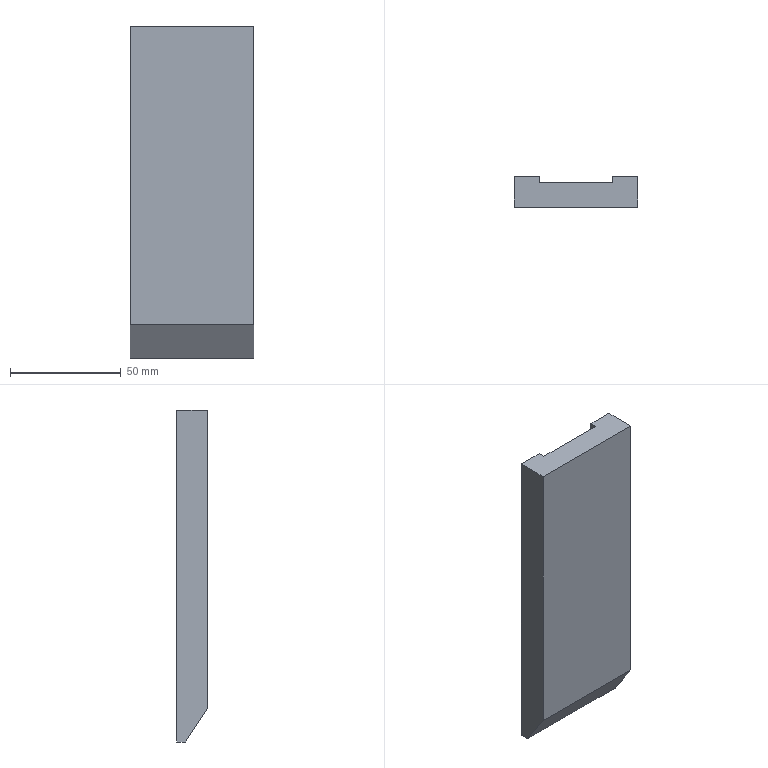Component | SolidWorks | CHEN123-AA-16-1 | 1 solid | 11 faces | box 56 x 14 x 150 mm | volume 98550 mm3 | plane 11
build123d program:
from build123d import *

# Parameters (mm, degrees)
SKETCH1_W           = 150
SKETCH1_H           = 56
BOSS_EXTRUDE1_DEPTH = 14
CUT_EXTRUDE1_DEPTH  = 95.641
SKETCH3_W           = 197.23
SKETCH3_H           = 33
CUT_EXTRUDE2_DEPTH  = 3


with BuildPart() as part:
    # Sketch1 → Boss-Extrude1 (new body)
    with BuildSketch(Plane.XY):
        Rectangle(SKETCH1_W, SKETCH1_H)
    extrude(amount=BOSS_EXTRUDE1_DEPTH)

    # Sketch2 → Cut-Extrude1 (cut, through all)
    with BuildSketch(Plane(origin=(0, 28, 0), x_dir=(1, 0, 0), z_dir=(0, 1, 0))):
        Polygon((-75, -14), (-75, -4), (-60, -14), align=None)
    extrude(amount=-CUT_EXTRUDE1_DEPTH, mode=Mode.SUBTRACT)

    # Sketch3 → Cut-Extrude2 (cut)
    with BuildSketch(Plane(origin=(0, 0, 0), x_dir=(-1, 0, 0), z_dir=(0, 0, -1))):
        Rectangle(SKETCH3_W, SKETCH3_H)
    extrude(amount=-CUT_EXTRUDE2_DEPTH, mode=Mode.SUBTRACT)


solid = part.part

# Placed as in the assembly
solid = solid.moved(Location((-0.0005, 34.001, -345), (90, 0, 90)))
STEP:
#1=CARTESIAN_POINT('',(-0.6496,1.339,-16.535));
#2=VERTEX_POINT('',#1);
#3=CARTESIAN_POINT('',(-0.6496,1.339,-10.63));
#4=VERTEX_POINT('',#3);
#5=CARTESIAN_POINT('',(-0.6496,1.339,-13.583));
#6=DIRECTION('',(0.,0.,1.));
#7=VECTOR('',#6,39.37);
#8=LINE('',#5,#7);
#9=EDGE_CURVE('',#2,#4,#8,.T.);
#10=ORIENTED_EDGE('',*,*,#9,.F.);
#11=CARTESIAN_POINT('',(-1.102,1.339,-16.535));
#12=VERTEX_POINT('',#11);
#13=CARTESIAN_POINT('',(1.102,1.339,-16.535));
#14=DIRECTION('',(1.,-0.,-0.));
#15=VECTOR('',#14,39.37);
#16=LINE('',#13,#15);
#17=EDGE_CURVE('',#12,#2,#16,.T.);
#18=ORIENTED_EDGE('',*,*,#17,.F.);
#19=CARTESIAN_POINT('',(-1.102,1.339,-10.63));
#20=VERTEX_POINT('',#19);
#21=CARTESIAN_POINT('',(-1.102,1.339,-16.535));
#22=DIRECTION('',(-0.,-0.,-1.));
#23=VECTOR('',#22,39.37);
#24=LINE('',#21,#23);
#25=EDGE_CURVE('',#20,#12,#24,.T.);
#26=ORIENTED_EDGE('',*,*,#25,.F.);
#27=CARTESIAN_POINT('',(1.102,1.339,-10.63));
#28=DIRECTION('',(-1.,0.,0.));
#29=VECTOR('',#28,39.37);
#30=LINE('',#27,#29);
#31=EDGE_CURVE('',#4,#20,#30,.T.);
#32=ORIENTED_EDGE('',*,*,#31,.F.);
#33=EDGE_LOOP('',(#10,#18,#26,#32));
#34=FACE_OUTER_BOUND('',#33,.T.);
#35=CARTESIAN_POINT('',(-0.00001969,1.339,-13.583));
#36=DIRECTION('',(0.,1.,-0.));
#37=DIRECTION('',(-0.,-0.,-1.));
#38=AXIS2_PLACEMENT_3D('',#35,#36,#37);
#39=PLANE('',#38);
#40=ADVANCED_FACE('',(#34),#39,.T.);
#41=CARTESIAN_POINT('',(0.6496,1.221,-10.63));
#42=VERTEX_POINT('',#41);
#43=CARTESIAN_POINT('',(-0.6496,1.221,-10.63));
#44=VERTEX_POINT('',#43);
#45=CARTESIAN_POINT('',(1.102,1.221,-10.63));
#46=DIRECTION('',(-1.,0.,0.));
#47=VECTOR('',#46,39.37);
#48=LINE('',#45,#47);
#49=EDGE_CURVE('',#42,#44,#48,.T.);
#50=ORIENTED_EDGE('',*,*,#49,.T.);
#51=CARTESIAN_POINT('',(-0.6496,0.7874,-10.63));
#52=DIRECTION('',(0.,1.,-0.));
#53=VECTOR('',#52,39.37);
#54=LINE('',#51,#53);
#55=EDGE_CURVE('',#44,#4,#54,.T.);
#56=ORIENTED_EDGE('',*,*,#55,.T.);
#57=ORIENTED_EDGE('',*,*,#31,.T.);
#58=CARTESIAN_POINT('',(-1.102,0.7874,-10.63));
#59=VERTEX_POINT('',#58);
#60=CARTESIAN_POINT('',(-1.102,0.7874,-10.63));
#61=DIRECTION('',(0.,1.,-0.));
#62=VECTOR('',#61,39.37);
#63=LINE('',#60,#62);
#64=EDGE_CURVE('',#59,#20,#63,.T.);
#65=ORIENTED_EDGE('',*,*,#64,.F.);
#66=CARTESIAN_POINT('',(1.102,0.7874,-10.63));
#67=VERTEX_POINT('',#66);
#68=CARTESIAN_POINT('',(1.102,0.7874,-10.63));
#69=DIRECTION('',(-1.,0.,0.));
#70=VECTOR('',#69,39.37);
#71=LINE('',#68,#70);
#72=EDGE_CURVE('',#67,#59,#71,.T.);
#73=ORIENTED_EDGE('',*,*,#72,.F.);
#74=CARTESIAN_POINT('',(1.102,1.339,-10.63));
#75=VERTEX_POINT('',#74);
#76=CARTESIAN_POINT('',(1.102,0.7874,-10.63));
#77=DIRECTION('',(0.,1.,-0.));
#78=VECTOR('',#77,39.37);
#79=LINE('',#76,#78);
#80=EDGE_CURVE('',#67,#75,#79,.T.);
#81=ORIENTED_EDGE('',*,*,#80,.T.);
#82=CARTESIAN_POINT('',(0.6496,1.339,-10.63));
#83=VERTEX_POINT('',#82);
#84=CARTESIAN_POINT('',(1.102,1.339,-10.63));
#85=DIRECTION('',(-1.,0.,0.));
#86=VECTOR('',#85,39.37);
#87=LINE('',#84,#86);
#88=EDGE_CURVE('',#75,#83,#87,.T.);
#89=ORIENTED_EDGE('',*,*,#88,.T.);
#90=CARTESIAN_POINT('',(0.6496,0.7874,-10.63));
#91=DIRECTION('',(-0.,-1.,0.));
#92=VECTOR('',#91,39.37);
#93=LINE('',#90,#92);
#94=EDGE_CURVE('',#83,#42,#93,.T.);
#95=ORIENTED_EDGE('',*,*,#94,.T.);
#96=EDGE_LOOP('',(#50,#56,#57,#65,#73,#81,#89,#95));
#97=FACE_OUTER_BOUND('',#96,.T.);
#98=CARTESIAN_POINT('',(1.102,0.7874,-10.63));
#99=DIRECTION('',(-0.,-0.,-1.));
#100=DIRECTION('',(-0.,-1.,0.));
#101=AXIS2_PLACEMENT_3D('',#98,#99,#100);
#102=PLANE('',#101);
#103=ADVANCED_FACE('',(#97),#102,.F.);
#104=CARTESIAN_POINT('',(-1.102,1.181,-16.535));
#105=VERTEX_POINT('',#104);
#106=CARTESIAN_POINT('',(-1.102,0.7874,-16.535));
#107=DIRECTION('',(0.,1.,-0.));
#108=VECTOR('',#107,39.37);
#109=LINE('',#106,#108);
#110=EDGE_CURVE('',#105,#12,#109,.T.);
#111=ORIENTED_EDGE('',*,*,#110,.F.);
#112=CARTESIAN_POINT('',(-1.102,0.7874,-15.945));
#113=VERTEX_POINT('',#112);
#114=CARTESIAN_POINT('',(-1.102,1.181,-16.535));
#115=DIRECTION('',(-0.,0.5547,-0.8321));
#116=VECTOR('',#115,39.37);
#117=LINE('',#114,#116);
#118=EDGE_CURVE('',#113,#105,#117,.T.);
#119=ORIENTED_EDGE('',*,*,#118,.F.);
#120=CARTESIAN_POINT('',(-1.102,0.7874,-16.535));
#121=DIRECTION('',(-0.,-0.,-1.));
#122=VECTOR('',#121,39.37);
#123=LINE('',#120,#122);
#124=EDGE_CURVE('',#59,#113,#123,.T.);
#125=ORIENTED_EDGE('',*,*,#124,.F.);
#126=ORIENTED_EDGE('',*,*,#64,.T.);
#127=ORIENTED_EDGE('',*,*,#25,.T.);
#128=EDGE_LOOP('',(#111,#119,#125,#126,#127));
#129=FACE_OUTER_BOUND('',#128,.T.);
#130=CARTESIAN_POINT('',(-1.102,0.7874,-16.535));
#131=DIRECTION('',(1.,-0.,-0.));
#132=DIRECTION('',(0.,1.,-0.));
#133=AXIS2_PLACEMENT_3D('',#130,#131,#132);
#134=PLANE('',#133);
#135=ADVANCED_FACE('',(#129),#134,.F.);
#136=ORIENTED_EDGE('',*,*,#17,.T.);
#137=CARTESIAN_POINT('',(-0.6496,1.221,-16.535));
#138=VERTEX_POINT('',#137);
#139=CARTESIAN_POINT('',(-0.6496,0.7874,-16.535));
#140=DIRECTION('',(-0.,-1.,0.));
#141=VECTOR('',#140,39.37);
#142=LINE('',#139,#141);
#143=EDGE_CURVE('',#2,#138,#142,.T.);
#144=ORIENTED_EDGE('',*,*,#143,.T.);
#145=CARTESIAN_POINT('',(0.6496,1.221,-16.535));
#146=VERTEX_POINT('',#145);
#147=CARTESIAN_POINT('',(1.102,1.221,-16.535));
#148=DIRECTION('',(1.,-0.,-0.));
#149=VECTOR('',#148,39.37);
#150=LINE('',#147,#149);
#151=EDGE_CURVE('',#138,#146,#150,.T.);
#152=ORIENTED_EDGE('',*,*,#151,.T.);
#153=CARTESIAN_POINT('',(0.6496,1.339,-16.535));
#154=VERTEX_POINT('',#153);
#155=CARTESIAN_POINT('',(0.6496,0.7874,-16.535));
#156=DIRECTION('',(0.,1.,-0.));
#157=VECTOR('',#156,39.37);
#158=LINE('',#155,#157);
#159=EDGE_CURVE('',#146,#154,#158,.T.);
#160=ORIENTED_EDGE('',*,*,#159,.T.);
#161=CARTESIAN_POINT('',(1.102,1.339,-16.535));
#162=VERTEX_POINT('',#161);
#163=CARTESIAN_POINT('',(1.102,1.339,-16.535));
#164=DIRECTION('',(1.,-0.,-0.));
#165=VECTOR('',#164,39.37);
#166=LINE('',#163,#165);
#167=EDGE_CURVE('',#154,#162,#166,.T.);
#168=ORIENTED_EDGE('',*,*,#167,.T.);
#169=CARTESIAN_POINT('',(1.102,1.181,-16.535));
#170=VERTEX_POINT('',#169);
#171=CARTESIAN_POINT('',(1.102,0.7874,-16.535));
#172=DIRECTION('',(0.,1.,-0.));
#173=VECTOR('',#172,39.37);
#174=LINE('',#171,#173);
#175=EDGE_CURVE('',#170,#162,#174,.T.);
#176=ORIENTED_EDGE('',*,*,#175,.F.);
#177=CARTESIAN_POINT('',(1.102,1.181,-16.535));
#178=DIRECTION('',(-1.,0.,0.));
#179=VECTOR('',#178,39.37);
#180=LINE('',#177,#179);
#181=EDGE_CURVE('',#170,#105,#180,.T.);
#182=ORIENTED_EDGE('',*,*,#181,.T.);
#183=ORIENTED_EDGE('',*,*,#110,.T.);
#184=EDGE_LOOP('',(#136,#144,#152,#160,#168,#176,#182,#183));
#185=FACE_OUTER_BOUND('',#184,.T.);
#186=CARTESIAN_POINT('',(1.102,0.7874,-16.535));
#187=DIRECTION('',(0.,0.,1.));
#188=DIRECTION('',(0.,1.,-0.));
#189=AXIS2_PLACEMENT_3D('',#186,#187,#188);
#190=PLANE('',#189);
#191=ADVANCED_FACE('',(#185),#190,.F.);
#192=CARTESIAN_POINT('',(1.102,0.7874,-15.945));
#193=VERTEX_POINT('',#192);
#194=CARTESIAN_POINT('',(1.102,0.7874,-16.535));
#195=DIRECTION('',(0.,0.,1.));
#196=VECTOR('',#195,39.37);
#197=LINE('',#194,#196);
#198=EDGE_CURVE('',#193,#67,#197,.T.);
#199=ORIENTED_EDGE('',*,*,#198,.F.);
#200=CARTESIAN_POINT('',(1.102,1.181,-16.535));
#201=DIRECTION('',(-0.,0.5547,-0.8321));
#202=VECTOR('',#201,39.37);
#203=LINE('',#200,#202);
#204=EDGE_CURVE('',#193,#170,#203,.T.);
#205=ORIENTED_EDGE('',*,*,#204,.T.);
#206=ORIENTED_EDGE('',*,*,#175,.T.);
#207=CARTESIAN_POINT('',(1.102,1.339,-16.535));
#208=DIRECTION('',(0.,0.,1.));
#209=VECTOR('',#208,39.37);
#210=LINE('',#207,#209);
#211=EDGE_CURVE('',#162,#75,#210,.T.);
#212=ORIENTED_EDGE('',*,*,#211,.T.);
#213=ORIENTED_EDGE('',*,*,#80,.F.);
#214=EDGE_LOOP('',(#199,#205,#206,#212,#213));
#215=FACE_OUTER_BOUND('',#214,.T.);
#216=CARTESIAN_POINT('',(1.102,0.7874,-16.535));
#217=DIRECTION('',(-1.,0.,0.));
#218=DIRECTION('',(-0.,-1.,0.));
#219=AXIS2_PLACEMENT_3D('',#216,#217,#218);
#220=PLANE('',#219);
#221=ADVANCED_FACE('',(#215),#220,.F.);
#222=ORIENTED_EDGE('',*,*,#124,.T.);
#223=CARTESIAN_POINT('',(1.102,0.7874,-15.945));
#224=DIRECTION('',(-1.,0.,0.));
#225=VECTOR('',#224,39.37);
#226=LINE('',#223,#225);
#227=EDGE_CURVE('',#193,#113,#226,.T.);
#228=ORIENTED_EDGE('',*,*,#227,.F.);
#229=ORIENTED_EDGE('',*,*,#198,.T.);
#230=ORIENTED_EDGE('',*,*,#72,.T.);
#231=EDGE_LOOP('',(#222,#228,#229,#230));
#232=FACE_OUTER_BOUND('',#231,.T.);
#233=CARTESIAN_POINT('',(-0.00001969,0.7874,-13.583));
#234=DIRECTION('',(0.,1.,-0.));
#235=DIRECTION('',(-0.,-0.,-1.));
#236=AXIS2_PLACEMENT_3D('',#233,#234,#235);
#237=PLANE('',#236);
#238=ADVANCED_FACE('',(#232),#237,.F.);
#239=CARTESIAN_POINT('',(0.6496,1.339,-13.583));
#240=DIRECTION('',(-0.,-0.,-1.));
#241=VECTOR('',#240,39.37);
#242=LINE('',#239,#241);
#243=EDGE_CURVE('',#83,#154,#242,.T.);
#244=ORIENTED_EDGE('',*,*,#243,.F.);
#245=ORIENTED_EDGE('',*,*,#88,.F.);
#246=ORIENTED_EDGE('',*,*,#211,.F.);
#247=ORIENTED_EDGE('',*,*,#167,.F.);
#248=EDGE_LOOP('',(#244,#245,#246,#247));
#249=FACE_OUTER_BOUND('',#248,.T.);
#250=CARTESIAN_POINT('',(-0.00001969,1.339,-13.583));
#251=DIRECTION('',(0.,1.,-0.));
#252=DIRECTION('',(-0.,-0.,-1.));
#253=AXIS2_PLACEMENT_3D('',#250,#251,#252);
#254=PLANE('',#253);
#255=ADVANCED_FACE('',(#249),#254,.T.);
#256=ORIENTED_EDGE('',*,*,#118,.T.);
#257=ORIENTED_EDGE('',*,*,#181,.F.);
#258=ORIENTED_EDGE('',*,*,#204,.F.);
#259=ORIENTED_EDGE('',*,*,#227,.T.);
#260=EDGE_LOOP('',(#256,#257,#258,#259));
#261=FACE_OUTER_BOUND('',#260,.T.);
#262=CARTESIAN_POINT('',(1.102,1.181,-16.535));
#263=DIRECTION('',(0.,0.8321,0.5547));
#264=DIRECTION('',(-0.,0.5547,-0.8321));
#265=AXIS2_PLACEMENT_3D('',#262,#263,#264);
#266=PLANE('',#265);
#267=ADVANCED_FACE('',(#261),#266,.F.);
#268=CARTESIAN_POINT('',(0.6496,1.221,-17.465));
#269=DIRECTION('',(-0.,-0.,-1.));
#270=VECTOR('',#269,39.37);
#271=LINE('',#268,#270);
#272=EDGE_CURVE('',#42,#146,#271,.T.);
#273=ORIENTED_EDGE('',*,*,#272,.T.);
#274=ORIENTED_EDGE('',*,*,#151,.F.);
#275=CARTESIAN_POINT('',(-0.6496,1.221,-17.465));
#276=DIRECTION('',(0.,0.,1.));
#277=VECTOR('',#276,39.37);
#278=LINE('',#275,#277);
#279=EDGE_CURVE('',#138,#44,#278,.T.);
#280=ORIENTED_EDGE('',*,*,#279,.T.);
#281=ORIENTED_EDGE('',*,*,#49,.F.);
#282=EDGE_LOOP('',(#273,#274,#280,#281));
#283=FACE_OUTER_BOUND('',#282,.T.);
#284=CARTESIAN_POINT('',(-0.00001969,1.221,-13.583));
#285=DIRECTION('',(-0.,-1.,0.));
#286=DIRECTION('',(0.,0.,1.));
#287=AXIS2_PLACEMENT_3D('',#284,#285,#286);
#288=PLANE('',#287);
#289=ADVANCED_FACE('',(#283),#288,.F.);
#290=ORIENTED_EDGE('',*,*,#279,.F.);
#291=ORIENTED_EDGE('',*,*,#143,.F.);
#292=ORIENTED_EDGE('',*,*,#9,.T.);
#293=ORIENTED_EDGE('',*,*,#55,.F.);
#294=EDGE_LOOP('',(#290,#291,#292,#293));
#295=FACE_OUTER_BOUND('',#294,.T.);
#296=CARTESIAN_POINT('',(-0.6496,1.221,-17.465));
#297=DIRECTION('',(-1.,0.,0.));
#298=DIRECTION('',(-0.,-0.,-1.));
#299=AXIS2_PLACEMENT_3D('',#296,#297,#298);
#300=PLANE('',#299);
#301=ADVANCED_FACE('',(#295),#300,.F.);
#302=ORIENTED_EDGE('',*,*,#243,.T.);
#303=ORIENTED_EDGE('',*,*,#159,.F.);
#304=ORIENTED_EDGE('',*,*,#272,.F.);
#305=ORIENTED_EDGE('',*,*,#94,.F.);
#306=EDGE_LOOP('',(#302,#303,#304,#305));
#307=FACE_OUTER_BOUND('',#306,.T.);
#308=CARTESIAN_POINT('',(0.6496,1.221,-17.465));
#309=DIRECTION('',(1.,-0.,-0.));
#310=DIRECTION('',(0.,0.,1.));
#311=AXIS2_PLACEMENT_3D('',#308,#309,#310);
#312=PLANE('',#311);
#313=ADVANCED_FACE('',(#307),#312,.F.);
#314=CLOSED_SHELL('',(#40,#103,#135,#191,#221,#238,#255,#267,#289,#301,#313));
#315=MANIFOLD_SOLID_BREP('',#314);
#316=CARTESIAN_POINT('',(0.,0.,0.));
#317=DIRECTION('',(0.,0.,1.));
#318=DIRECTION('',(1.,0.,0.));
#319=AXIS2_PLACEMENT_3D('',#316,#317,#318);
#320=(LENGTH_UNIT()NAMED_UNIT(*)SI_UNIT($,.METRE.));
#321=LENGTH_MEASURE_WITH_UNIT(LENGTH_MEASURE(0.0254),#320);
#322=DIMENSIONAL_EXPONENTS(1.,0.,0.,0.,0.,0.,0.);
#323=(CONVERSION_BASED_UNIT('',#321)LENGTH_UNIT()NAMED_UNIT(#322));
#324=UNCERTAINTY_MEASURE_WITH_UNIT(LENGTH_MEASURE(0.00001),#323,'','');
#325=(NAMED_UNIT(*)PLANE_ANGLE_UNIT()SI_UNIT($,.RADIAN.));
#326=(NAMED_UNIT(*)SI_UNIT($,.STERADIAN.)SOLID_ANGLE_UNIT());
#327=(GEOMETRIC_REPRESENTATION_CONTEXT(3)GLOBAL_UNCERTAINTY_ASSIGNED_CONTEXT((#324))GLOBAL_UNIT_ASSIGNED_CONTEXT((#323,#325,#326))REPRESENTATION_CONTEXT('',''));
#328=ADVANCED_BREP_SHAPE_REPRESENTATION('',(#315,#319),#327);
#329=COLOUR_RGB('',0.7922,0.8196,0.9333);
#330=FILL_AREA_STYLE_COLOUR('',#329);
#331=FILL_AREA_STYLE('',(#330));
#332=SURFACE_STYLE_FILL_AREA(#331);
#333=SURFACE_SIDE_STYLE('',(#332));
#334=SURFACE_STYLE_USAGE(.BOTH.,#333);
#335=PRESENTATION_STYLE_ASSIGNMENT((#334));
#336=STYLED_ITEM('',(#335),#315);
#337=PRESENTATION_LAYER_ASSIGNMENT('','',(#336));
#338=(LENGTH_UNIT()NAMED_UNIT(*)SI_UNIT($,.METRE.));
#339=LENGTH_MEASURE_WITH_UNIT(LENGTH_MEASURE(0.0254),#338);
#340=DIMENSIONAL_EXPONENTS(1.,0.,0.,0.,0.,0.,0.);
#341=(CONVERSION_BASED_UNIT('',#339)LENGTH_UNIT()NAMED_UNIT(#340));
#342=UNCERTAINTY_MEASURE_WITH_UNIT(LENGTH_MEASURE(0.00001),#341,'','');
#343=(NAMED_UNIT(*)PLANE_ANGLE_UNIT()SI_UNIT($,.RADIAN.));
#344=(NAMED_UNIT(*)SI_UNIT($,.STERADIAN.)SOLID_ANGLE_UNIT());
#345=(GEOMETRIC_REPRESENTATION_CONTEXT(3)GLOBAL_UNCERTAINTY_ASSIGNED_CONTEXT((#342))GLOBAL_UNIT_ASSIGNED_CONTEXT((#341,#343,#344))REPRESENTATION_CONTEXT('',''));
#346=MECHANICAL_DESIGN_GEOMETRIC_PRESENTATION_REPRESENTATION('',(#336),#345);